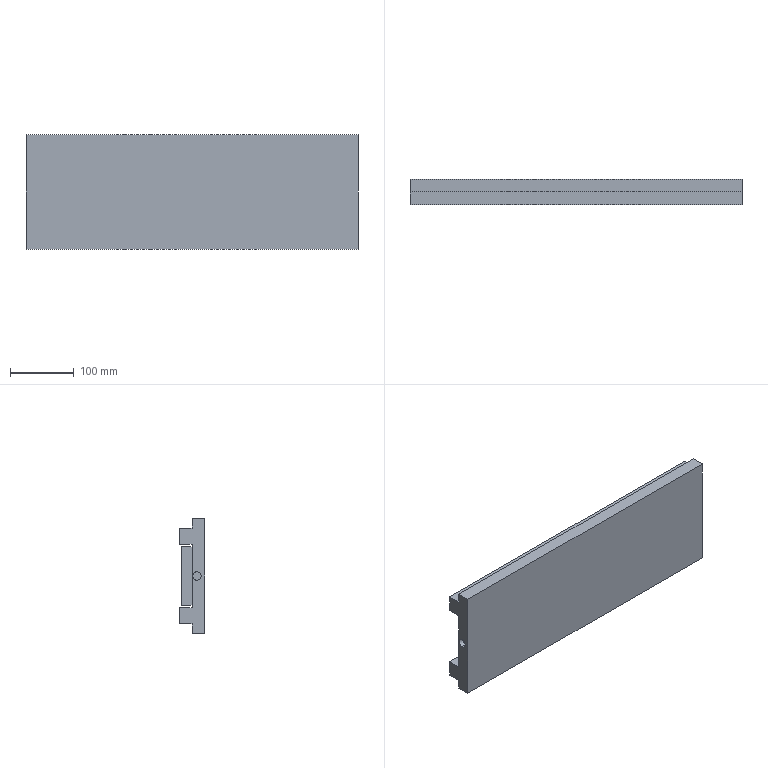Component | SolidWorks | X-AxisSupportBase-1 | 1 solid | 41 faces | volume 2443332 mm3 | plane 28 | cylinder 13 | commonest cylinder face diameters 5.084 x8 13.093 x2 2.946 x2 49.2 x1